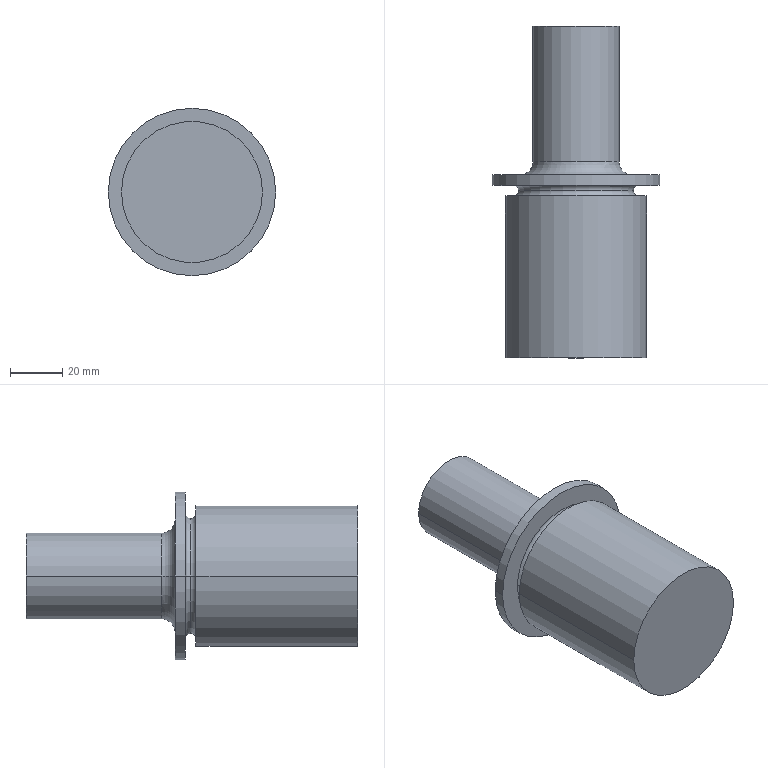Component | SolidWorks | Assembly4.1-1_114.1-1 | 1 solid | 17 faces | box 64 x 127 x 64 mm | volume 210532 mm3 | torus 6 | cylinder 6 | plane 5 | commonest cylinder face diameters 54 x2 64 x2 33 x2
STEP:
#1=CARTESIAN_POINT('',(-0.9449,-1.555,-0.01575));
#2=VERTEX_POINT('',#1);
#3=CARTESIAN_POINT('',(0.9449,-1.555,-0.01575));
#4=VERTEX_POINT('',#3);
#5=CARTESIAN_POINT('',(-0.,-1.555,-0.01575));
#6=DIRECTION('',(-0.,-1.,0.));
#7=DIRECTION('',(1.,0.,0.));
#8=AXIS2_PLACEMENT_3D('',#5,#6,#7);
#9=CIRCLE('',#8,0.9449);
#10=EDGE_CURVE('',#2,#4,#9,.T.);
#11=ORIENTED_EDGE('',*,*,#10,.F.);
#12=CARTESIAN_POINT('',(-0.8661,-1.476,-0.01575));
#13=VERTEX_POINT('',#12);
#14=CARTESIAN_POINT('',(-0.9449,-1.476,-0.01575));
#15=DIRECTION('',(-0.,0.,1.));
#16=DIRECTION('',(1.,0.,0.));
#17=AXIS2_PLACEMENT_3D('',#14,#15,#16);
#18=CIRCLE('',#17,0.07874);
#19=EDGE_CURVE('',#2,#13,#18,.T.);
#20=ORIENTED_EDGE('',*,*,#19,.T.);
#21=CARTESIAN_POINT('',(0.8661,-1.476,-0.01575));
#22=VERTEX_POINT('',#21);
#23=CARTESIAN_POINT('',(-0.,-1.476,-0.01575));
#24=DIRECTION('',(-0.,-1.,0.));
#25=DIRECTION('',(1.,0.,0.));
#26=AXIS2_PLACEMENT_3D('',#23,#24,#25);
#27=CIRCLE('',#26,0.8661);
#28=EDGE_CURVE('',#13,#22,#27,.T.);
#29=ORIENTED_EDGE('',*,*,#28,.T.);
#30=CARTESIAN_POINT('',(0.9449,-1.476,-0.01575));
#31=DIRECTION('',(0.,-0.,-1.));
#32=DIRECTION('',(-1.,0.,-0.));
#33=AXIS2_PLACEMENT_3D('',#30,#31,#32);
#34=CIRCLE('',#33,0.07874);
#35=EDGE_CURVE('',#4,#22,#34,.T.);
#36=ORIENTED_EDGE('',*,*,#35,.F.);
#37=EDGE_LOOP('',(#11,#20,#29,#36));
#38=FACE_OUTER_BOUND('',#37,.T.);
#39=CARTESIAN_POINT('',(-0.,-1.476,-0.01575));
#40=DIRECTION('',(-0.,-1.,0.));
#41=DIRECTION('',(1.,-0.,0.));
#42=AXIS2_PLACEMENT_3D('',#39,#40,#41);
#43=TOROIDAL_SURFACE('',#42,0.9449,0.07874);
#44=ADVANCED_FACE('',(#38),#43,.F.);
#45=ORIENTED_EDGE('',*,*,#28,.F.);
#46=CARTESIAN_POINT('',(-0.9449,-1.398,-0.01575));
#47=VERTEX_POINT('',#46);
#48=CARTESIAN_POINT('',(-0.9449,-1.476,-0.01575));
#49=DIRECTION('',(-0.,0.,1.));
#50=DIRECTION('',(1.,0.,0.));
#51=AXIS2_PLACEMENT_3D('',#48,#49,#50);
#52=CIRCLE('',#51,0.07874);
#53=EDGE_CURVE('',#13,#47,#52,.T.);
#54=ORIENTED_EDGE('',*,*,#53,.T.);
#55=CARTESIAN_POINT('',(0.9449,-1.398,-0.01575));
#56=VERTEX_POINT('',#55);
#57=CARTESIAN_POINT('',(-0.,-1.398,-0.01575));
#58=DIRECTION('',(0.,1.,-0.));
#59=DIRECTION('',(1.,0.,0.));
#60=AXIS2_PLACEMENT_3D('',#57,#58,#59);
#61=CIRCLE('',#60,0.9449);
#62=EDGE_CURVE('',#56,#47,#61,.T.);
#63=ORIENTED_EDGE('',*,*,#62,.F.);
#64=CARTESIAN_POINT('',(0.9449,-1.476,-0.01575));
#65=DIRECTION('',(0.,-0.,-1.));
#66=DIRECTION('',(-1.,0.,-0.));
#67=AXIS2_PLACEMENT_3D('',#64,#65,#66);
#68=CIRCLE('',#67,0.07874);
#69=EDGE_CURVE('',#22,#56,#68,.T.);
#70=ORIENTED_EDGE('',*,*,#69,.F.);
#71=EDGE_LOOP('',(#45,#54,#63,#70));
#72=FACE_OUTER_BOUND('',#71,.T.);
#73=CARTESIAN_POINT('',(-0.,-1.476,-0.01575));
#74=DIRECTION('',(-0.,-1.,0.));
#75=DIRECTION('',(1.,-0.,0.));
#76=AXIS2_PLACEMENT_3D('',#73,#74,#75);
#77=TOROIDAL_SURFACE('',#76,0.9449,0.07874);
#78=ADVANCED_FACE('',(#72),#77,.F.);
#79=CARTESIAN_POINT('',(1.063,-3.996,-0.01575));
#80=VERTEX_POINT('',#79);
#81=CARTESIAN_POINT('',(-1.063,-3.996,-0.01575));
#82=VERTEX_POINT('',#81);
#83=CARTESIAN_POINT('',(-0.,-3.996,-0.01575));
#84=DIRECTION('',(-0.,-1.,0.));
#85=DIRECTION('',(1.,0.,0.));
#86=AXIS2_PLACEMENT_3D('',#83,#84,#85);
#87=CIRCLE('',#86,1.063);
#88=EDGE_CURVE('',#80,#82,#87,.T.);
#89=ORIENTED_EDGE('',*,*,#88,.F.);
#90=CARTESIAN_POINT('',(1.063,-1.555,-0.01575));
#91=VERTEX_POINT('',#90);
#92=CARTESIAN_POINT('',(1.063,-3.996,-0.01575));
#93=DIRECTION('',(0.,1.,-0.));
#94=VECTOR('',#93,39.37);
#95=LINE('',#92,#94);
#96=EDGE_CURVE('',#80,#91,#95,.T.);
#97=ORIENTED_EDGE('',*,*,#96,.T.);
#98=CARTESIAN_POINT('',(-1.063,-1.555,-0.01575));
#99=VERTEX_POINT('',#98);
#100=CARTESIAN_POINT('',(-0.,-1.555,-0.01575));
#101=DIRECTION('',(-0.,-1.,0.));
#102=DIRECTION('',(1.,0.,0.));
#103=AXIS2_PLACEMENT_3D('',#100,#101,#102);
#104=CIRCLE('',#103,1.063);
#105=EDGE_CURVE('',#91,#99,#104,.T.);
#106=ORIENTED_EDGE('',*,*,#105,.T.);
#107=CARTESIAN_POINT('',(-1.063,-3.996,-0.01575));
#108=DIRECTION('',(0.,1.,-0.));
#109=VECTOR('',#108,39.37);
#110=LINE('',#107,#109);
#111=EDGE_CURVE('',#82,#99,#110,.T.);
#112=ORIENTED_EDGE('',*,*,#111,.F.);
#113=EDGE_LOOP('',(#89,#97,#106,#112));
#114=FACE_OUTER_BOUND('',#113,.T.);
#115=CARTESIAN_POINT('',(-0.,-3.996,-0.01575));
#116=DIRECTION('',(0.,1.,-0.));
#117=DIRECTION('',(-1.,0.,-0.));
#118=AXIS2_PLACEMENT_3D('',#115,#116,#117);
#119=CYLINDRICAL_SURFACE('',#118,1.063);
#120=ADVANCED_FACE('',(#114),#119,.T.);
#121=CARTESIAN_POINT('',(-0.8465,-1.24,-0.01575));
#122=VERTEX_POINT('',#121);
#123=CARTESIAN_POINT('',(0.8465,-1.24,-0.01575));
#124=VERTEX_POINT('',#123);
#125=CARTESIAN_POINT('',(-0.,-1.24,-0.01575));
#126=DIRECTION('',(-0.,-1.,0.));
#127=DIRECTION('',(1.,0.,0.));
#128=AXIS2_PLACEMENT_3D('',#125,#126,#127);
#129=CIRCLE('',#128,0.8465);
#130=EDGE_CURVE('',#122,#124,#129,.T.);
#131=ORIENTED_EDGE('',*,*,#130,.F.);
#132=CARTESIAN_POINT('',(-0.6496,-1.043,-0.01575));
#133=VERTEX_POINT('',#132);
#134=CARTESIAN_POINT('',(-0.8465,-1.043,-0.01575));
#135=DIRECTION('',(-0.,0.,1.));
#136=DIRECTION('',(1.,0.,0.));
#137=AXIS2_PLACEMENT_3D('',#134,#135,#136);
#138=CIRCLE('',#137,0.1969);
#139=EDGE_CURVE('',#122,#133,#138,.T.);
#140=ORIENTED_EDGE('',*,*,#139,.T.);
#141=CARTESIAN_POINT('',(0.6496,-1.043,-0.01575));
#142=VERTEX_POINT('',#141);
#143=CARTESIAN_POINT('',(-0.,-1.043,-0.01575));
#144=DIRECTION('',(0.,1.,-0.));
#145=DIRECTION('',(1.,0.,0.));
#146=AXIS2_PLACEMENT_3D('',#143,#144,#145);
#147=CIRCLE('',#146,0.6496);
#148=EDGE_CURVE('',#142,#133,#147,.T.);
#149=ORIENTED_EDGE('',*,*,#148,.F.);
#150=CARTESIAN_POINT('',(0.8465,-1.043,-0.01575));
#151=DIRECTION('',(0.,-0.,-1.));
#152=DIRECTION('',(-1.,0.,-0.));
#153=AXIS2_PLACEMENT_3D('',#150,#151,#152);
#154=CIRCLE('',#153,0.1969);
#155=EDGE_CURVE('',#124,#142,#154,.T.);
#156=ORIENTED_EDGE('',*,*,#155,.F.);
#157=EDGE_LOOP('',(#131,#140,#149,#156));
#158=FACE_OUTER_BOUND('',#157,.T.);
#159=CARTESIAN_POINT('',(-0.,-1.043,-0.01575));
#160=DIRECTION('',(-0.,-1.,0.));
#161=DIRECTION('',(1.,-0.,0.));
#162=AXIS2_PLACEMENT_3D('',#159,#160,#161);
#163=TOROIDAL_SURFACE('',#162,0.8465,0.1969);
#164=ADVANCED_FACE('',(#158),#163,.F.);
#165=CARTESIAN_POINT('',(1.26,-1.398,-0.01575));
#166=VERTEX_POINT('',#165);
#167=CARTESIAN_POINT('',(-1.26,-1.398,-0.01575));
#168=VERTEX_POINT('',#167);
#169=CARTESIAN_POINT('',(-0.,-1.398,-0.01575));
#170=DIRECTION('',(-0.,-1.,0.));
#171=DIRECTION('',(1.,0.,0.));
#172=AXIS2_PLACEMENT_3D('',#169,#170,#171);
#173=CIRCLE('',#172,1.26);
#174=EDGE_CURVE('',#166,#168,#173,.T.);
#175=ORIENTED_EDGE('',*,*,#174,.F.);
#176=CARTESIAN_POINT('',(1.26,-1.24,-0.01575));
#177=VERTEX_POINT('',#176);
#178=CARTESIAN_POINT('',(1.26,-1.398,-0.01575));
#179=DIRECTION('',(0.,1.,-0.));
#180=VECTOR('',#179,39.37);
#181=LINE('',#178,#180);
#182=EDGE_CURVE('',#166,#177,#181,.T.);
#183=ORIENTED_EDGE('',*,*,#182,.T.);
#184=CARTESIAN_POINT('',(-1.26,-1.24,-0.01575));
#185=VERTEX_POINT('',#184);
#186=CARTESIAN_POINT('',(-0.,-1.24,-0.01575));
#187=DIRECTION('',(-0.,-1.,0.));
#188=DIRECTION('',(1.,0.,0.));
#189=AXIS2_PLACEMENT_3D('',#186,#187,#188);
#190=CIRCLE('',#189,1.26);
#191=EDGE_CURVE('',#177,#185,#190,.T.);
#192=ORIENTED_EDGE('',*,*,#191,.T.);
#193=CARTESIAN_POINT('',(-1.26,-1.398,-0.01575));
#194=DIRECTION('',(0.,1.,-0.));
#195=VECTOR('',#194,39.37);
#196=LINE('',#193,#195);
#197=EDGE_CURVE('',#168,#185,#196,.T.);
#198=ORIENTED_EDGE('',*,*,#197,.F.);
#199=EDGE_LOOP('',(#175,#183,#192,#198));
#200=FACE_OUTER_BOUND('',#199,.T.);
#201=CARTESIAN_POINT('',(-0.,-1.398,-0.01575));
#202=DIRECTION('',(0.,1.,-0.));
#203=DIRECTION('',(-1.,0.,-0.));
#204=AXIS2_PLACEMENT_3D('',#201,#202,#203);
#205=CYLINDRICAL_SURFACE('',#204,1.26);
#206=ADVANCED_FACE('',(#200),#205,.T.);
#207=CARTESIAN_POINT('',(-0.6496,1.004,-0.01575));
#208=VERTEX_POINT('',#207);
#209=CARTESIAN_POINT('',(0.6496,1.004,-0.01575));
#210=VERTEX_POINT('',#209);
#211=CARTESIAN_POINT('',(0.,1.004,-0.01575));
#212=DIRECTION('',(0.,1.,-0.));
#213=DIRECTION('',(-1.,0.,-0.));
#214=AXIS2_PLACEMENT_3D('',#211,#212,#213);
#215=CIRCLE('',#214,0.6496);
#216=EDGE_CURVE('',#208,#210,#215,.T.);
#217=ORIENTED_EDGE('',*,*,#216,.F.);
#218=CARTESIAN_POINT('',(-0.6496,1.004,-0.01575));
#219=DIRECTION('',(-0.,-1.,0.));
#220=VECTOR('',#219,39.37);
#221=LINE('',#218,#220);
#222=EDGE_CURVE('',#208,#133,#221,.T.);
#223=ORIENTED_EDGE('',*,*,#222,.T.);
#224=CARTESIAN_POINT('',(-0.,-1.043,-0.01575));
#225=DIRECTION('',(0.,1.,-0.));
#226=DIRECTION('',(1.,0.,0.));
#227=AXIS2_PLACEMENT_3D('',#224,#225,#226);
#228=CIRCLE('',#227,0.6496);
#229=EDGE_CURVE('',#133,#142,#228,.T.);
#230=ORIENTED_EDGE('',*,*,#229,.T.);
#231=CARTESIAN_POINT('',(0.6496,1.004,-0.01575));
#232=DIRECTION('',(-0.,-1.,0.));
#233=VECTOR('',#232,39.37);
#234=LINE('',#231,#233);
#235=EDGE_CURVE('',#210,#142,#234,.T.);
#236=ORIENTED_EDGE('',*,*,#235,.F.);
#237=EDGE_LOOP('',(#217,#223,#230,#236));
#238=FACE_OUTER_BOUND('',#237,.T.);
#239=CARTESIAN_POINT('',(0.,1.004,-0.01575));
#240=DIRECTION('',(-0.,-1.,0.));
#241=DIRECTION('',(1.,0.,0.));
#242=AXIS2_PLACEMENT_3D('',#239,#240,#241);
#243=CYLINDRICAL_SURFACE('',#242,0.6496);
#244=ADVANCED_FACE('',(#238),#243,.T.);
#245=ORIENTED_EDGE('',*,*,#62,.T.);
#246=CARTESIAN_POINT('',(-0.,-1.398,-0.01575));
#247=DIRECTION('',(0.,1.,-0.));
#248=DIRECTION('',(1.,0.,0.));
#249=AXIS2_PLACEMENT_3D('',#246,#247,#248);
#250=CIRCLE('',#249,0.9449);
#251=EDGE_CURVE('',#47,#56,#250,.T.);
#252=ORIENTED_EDGE('',*,*,#251,.T.);
#253=EDGE_LOOP('',(#245,#252));
#254=FACE_BOUND('',#253,.T.);
#255=CARTESIAN_POINT('',(-0.,-1.398,-0.01575));
#256=DIRECTION('',(-0.,-1.,0.));
#257=DIRECTION('',(1.,0.,0.));
#258=AXIS2_PLACEMENT_3D('',#255,#256,#257);
#259=CIRCLE('',#258,1.26);
#260=EDGE_CURVE('',#168,#166,#259,.T.);
#261=ORIENTED_EDGE('',*,*,#260,.T.);
#262=ORIENTED_EDGE('',*,*,#174,.T.);
#263=EDGE_LOOP('',(#261,#262));
#264=FACE_OUTER_BOUND('',#263,.T.);
#265=CARTESIAN_POINT('',(-0.,-1.398,-0.01575));
#266=DIRECTION('',(-0.,-1.,0.));
#267=DIRECTION('',(1.,-0.,0.));
#268=AXIS2_PLACEMENT_3D('',#265,#266,#267);
#269=PLANE('',#268);
#270=ADVANCED_FACE('',(#254,#264),#269,.T.);
#271=ORIENTED_EDGE('',*,*,#222,.F.);
#272=CARTESIAN_POINT('',(0.,1.004,-0.01575));
#273=DIRECTION('',(0.,1.,-0.));
#274=DIRECTION('',(-1.,0.,-0.));
#275=AXIS2_PLACEMENT_3D('',#272,#273,#274);
#276=CIRCLE('',#275,0.6496);
#277=EDGE_CURVE('',#210,#208,#276,.T.);
#278=ORIENTED_EDGE('',*,*,#277,.F.);
#279=ORIENTED_EDGE('',*,*,#235,.T.);
#280=ORIENTED_EDGE('',*,*,#148,.T.);
#281=EDGE_LOOP('',(#271,#278,#279,#280));
#282=FACE_OUTER_BOUND('',#281,.T.);
#283=CARTESIAN_POINT('',(0.,1.004,-0.01575));
#284=DIRECTION('',(-0.,-1.,0.));
#285=DIRECTION('',(1.,0.,0.));
#286=AXIS2_PLACEMENT_3D('',#283,#284,#285);
#287=CYLINDRICAL_SURFACE('',#286,0.6496);
#288=ADVANCED_FACE('',(#282),#287,.T.);
#289=ORIENTED_EDGE('',*,*,#277,.T.);
#290=ORIENTED_EDGE('',*,*,#216,.T.);
#291=EDGE_LOOP('',(#289,#290));
#292=FACE_OUTER_BOUND('',#291,.T.);
#293=CARTESIAN_POINT('',(0.,1.004,-0.01575));
#294=DIRECTION('',(0.,1.,-0.));
#295=DIRECTION('',(-1.,0.,-0.));
#296=AXIS2_PLACEMENT_3D('',#293,#294,#295);
#297=PLANE('',#296);
#298=ADVANCED_FACE('',(#292),#297,.T.);
#299=CARTESIAN_POINT('',(-0.,-1.24,-0.01575));
#300=DIRECTION('',(-0.,-1.,0.));
#301=DIRECTION('',(1.,0.,0.));
#302=AXIS2_PLACEMENT_3D('',#299,#300,#301);
#303=CIRCLE('',#302,0.8465);
#304=EDGE_CURVE('',#124,#122,#303,.T.);
#305=ORIENTED_EDGE('',*,*,#304,.T.);
#306=ORIENTED_EDGE('',*,*,#130,.T.);
#307=EDGE_LOOP('',(#305,#306));
#308=FACE_BOUND('',#307,.T.);
#309=CARTESIAN_POINT('',(-0.,-1.24,-0.01575));
#310=DIRECTION('',(-0.,-1.,0.));
#311=DIRECTION('',(1.,0.,0.));
#312=AXIS2_PLACEMENT_3D('',#309,#310,#311);
#313=CIRCLE('',#312,1.26);
#314=EDGE_CURVE('',#185,#177,#313,.T.);
#315=ORIENTED_EDGE('',*,*,#314,.F.);
#316=ORIENTED_EDGE('',*,*,#191,.F.);
#317=EDGE_LOOP('',(#315,#316));
#318=FACE_OUTER_BOUND('',#317,.T.);
#319=CARTESIAN_POINT('',(-0.,-1.24,-0.01575));
#320=DIRECTION('',(-0.,-1.,0.));
#321=DIRECTION('',(1.,-0.,0.));
#322=AXIS2_PLACEMENT_3D('',#319,#320,#321);
#323=PLANE('',#322);
#324=ADVANCED_FACE('',(#308,#318),#323,.F.);
#325=ORIENTED_EDGE('',*,*,#182,.F.);
#326=ORIENTED_EDGE('',*,*,#260,.F.);
#327=ORIENTED_EDGE('',*,*,#197,.T.);
#328=ORIENTED_EDGE('',*,*,#314,.T.);
#329=EDGE_LOOP('',(#325,#326,#327,#328));
#330=FACE_OUTER_BOUND('',#329,.T.);
#331=CARTESIAN_POINT('',(-0.,-1.398,-0.01575));
#332=DIRECTION('',(0.,1.,-0.));
#333=DIRECTION('',(-1.,0.,-0.));
#334=AXIS2_PLACEMENT_3D('',#331,#332,#333);
#335=CYLINDRICAL_SURFACE('',#334,1.26);
#336=ADVANCED_FACE('',(#330),#335,.T.);
#337=ORIENTED_EDGE('',*,*,#139,.F.);
#338=ORIENTED_EDGE('',*,*,#304,.F.);
#339=ORIENTED_EDGE('',*,*,#155,.T.);
#340=ORIENTED_EDGE('',*,*,#229,.F.);
#341=EDGE_LOOP('',(#337,#338,#339,#340));
#342=FACE_OUTER_BOUND('',#341,.T.);
#343=CARTESIAN_POINT('',(-0.,-1.043,-0.01575));
#344=DIRECTION('',(-0.,-1.,0.));
#345=DIRECTION('',(1.,-0.,0.));
#346=AXIS2_PLACEMENT_3D('',#343,#344,#345);
#347=TOROIDAL_SURFACE('',#346,0.8465,0.1969);
#348=ADVANCED_FACE('',(#342),#347,.F.);
#349=CARTESIAN_POINT('',(-0.,-1.555,-0.01575));
#350=DIRECTION('',(-0.,-1.,0.));
#351=DIRECTION('',(1.,0.,0.));
#352=AXIS2_PLACEMENT_3D('',#349,#350,#351);
#353=CIRCLE('',#352,0.9449);
#354=EDGE_CURVE('',#4,#2,#353,.T.);
#355=ORIENTED_EDGE('',*,*,#354,.T.);
#356=ORIENTED_EDGE('',*,*,#10,.T.);
#357=EDGE_LOOP('',(#355,#356));
#358=FACE_BOUND('',#357,.T.);
#359=CARTESIAN_POINT('',(-0.,-1.555,-0.01575));
#360=DIRECTION('',(-0.,-1.,0.));
#361=DIRECTION('',(1.,0.,0.));
#362=AXIS2_PLACEMENT_3D('',#359,#360,#361);
#363=CIRCLE('',#362,1.063);
#364=EDGE_CURVE('',#99,#91,#363,.T.);
#365=ORIENTED_EDGE('',*,*,#364,.F.);
#366=ORIENTED_EDGE('',*,*,#105,.F.);
#367=EDGE_LOOP('',(#365,#366));
#368=FACE_OUTER_BOUND('',#367,.T.);
#369=CARTESIAN_POINT('',(-0.,-1.555,-0.01575));
#370=DIRECTION('',(-0.,-1.,0.));
#371=DIRECTION('',(1.,-0.,0.));
#372=AXIS2_PLACEMENT_3D('',#369,#370,#371);
#373=PLANE('',#372);
#374=ADVANCED_FACE('',(#358,#368),#373,.F.);
#375=ORIENTED_EDGE('',*,*,#96,.F.);
#376=CARTESIAN_POINT('',(-0.,-3.996,-0.01575));
#377=DIRECTION('',(-0.,-1.,0.));
#378=DIRECTION('',(1.,0.,0.));
#379=AXIS2_PLACEMENT_3D('',#376,#377,#378);
#380=CIRCLE('',#379,1.063);
#381=EDGE_CURVE('',#82,#80,#380,.T.);
#382=ORIENTED_EDGE('',*,*,#381,.F.);
#383=ORIENTED_EDGE('',*,*,#111,.T.);
#384=ORIENTED_EDGE('',*,*,#364,.T.);
#385=EDGE_LOOP('',(#375,#382,#383,#384));
#386=FACE_OUTER_BOUND('',#385,.T.);
#387=CARTESIAN_POINT('',(-0.,-3.996,-0.01575));
#388=DIRECTION('',(0.,1.,-0.));
#389=DIRECTION('',(-1.,0.,-0.));
#390=AXIS2_PLACEMENT_3D('',#387,#388,#389);
#391=CYLINDRICAL_SURFACE('',#390,1.063);
#392=ADVANCED_FACE('',(#386),#391,.T.);
#393=ORIENTED_EDGE('',*,*,#381,.T.);
#394=ORIENTED_EDGE('',*,*,#88,.T.);
#395=EDGE_LOOP('',(#393,#394));
#396=FACE_OUTER_BOUND('',#395,.T.);
#397=CARTESIAN_POINT('',(-0.,-3.996,-0.01575));
#398=DIRECTION('',(-0.,-1.,0.));
#399=DIRECTION('',(1.,-0.,0.));
#400=AXIS2_PLACEMENT_3D('',#397,#398,#399);
#401=PLANE('',#400);
#402=ADVANCED_FACE('',(#396),#401,.T.);
#403=ORIENTED_EDGE('',*,*,#53,.F.);
#404=CARTESIAN_POINT('',(-0.,-1.476,-0.01575));
#405=DIRECTION('',(-0.,-1.,0.));
#406=DIRECTION('',(1.,0.,0.));
#407=AXIS2_PLACEMENT_3D('',#404,#405,#406);
#408=CIRCLE('',#407,0.8661);
#409=EDGE_CURVE('',#22,#13,#408,.T.);
#410=ORIENTED_EDGE('',*,*,#409,.F.);
#411=ORIENTED_EDGE('',*,*,#69,.T.);
#412=ORIENTED_EDGE('',*,*,#251,.F.);
#413=EDGE_LOOP('',(#403,#410,#411,#412));
#414=FACE_OUTER_BOUND('',#413,.T.);
#415=CARTESIAN_POINT('',(-0.,-1.476,-0.01575));
#416=DIRECTION('',(-0.,-1.,0.));
#417=DIRECTION('',(1.,-0.,0.));
#418=AXIS2_PLACEMENT_3D('',#415,#416,#417);
#419=TOROIDAL_SURFACE('',#418,0.9449,0.07874);
#420=ADVANCED_FACE('',(#414),#419,.F.);
#421=ORIENTED_EDGE('',*,*,#19,.F.);
#422=ORIENTED_EDGE('',*,*,#354,.F.);
#423=ORIENTED_EDGE('',*,*,#35,.T.);
#424=ORIENTED_EDGE('',*,*,#409,.T.);
#425=EDGE_LOOP('',(#421,#422,#423,#424));
#426=FACE_OUTER_BOUND('',#425,.T.);
#427=CARTESIAN_POINT('',(-0.,-1.476,-0.01575));
#428=DIRECTION('',(-0.,-1.,0.));
#429=DIRECTION('',(1.,-0.,0.));
#430=AXIS2_PLACEMENT_3D('',#427,#428,#429);
#431=TOROIDAL_SURFACE('',#430,0.9449,0.07874);
#432=ADVANCED_FACE('',(#426),#431,.F.);
#433=CLOSED_SHELL('',(#44,#78,#120,#164,#206,#244,#270,#288,#298,#324,#336,#348,#374,#392,#402,#420,#432));
#434=MANIFOLD_SOLID_BREP('',#433);
#435=CARTESIAN_POINT('',(0.,0.,0.));
#436=DIRECTION('',(0.,0.,1.));
#437=DIRECTION('',(1.,0.,0.));
#438=AXIS2_PLACEMENT_3D('',#435,#436,#437);
#439=(LENGTH_UNIT()NAMED_UNIT(*)SI_UNIT($,.METRE.));
#440=LENGTH_MEASURE_WITH_UNIT(LENGTH_MEASURE(0.0254),#439);
#441=DIMENSIONAL_EXPONENTS(1.,0.,0.,0.,0.,0.,0.);
#442=(CONVERSION_BASED_UNIT('',#440)LENGTH_UNIT()NAMED_UNIT(#441));
#443=UNCERTAINTY_MEASURE_WITH_UNIT(LENGTH_MEASURE(0.00001),#442,'','');
#444=(NAMED_UNIT(*)PLANE_ANGLE_UNIT()SI_UNIT($,.RADIAN.));
#445=(NAMED_UNIT(*)SI_UNIT($,.STERADIAN.)SOLID_ANGLE_UNIT());
#446=(GEOMETRIC_REPRESENTATION_CONTEXT(3)GLOBAL_UNCERTAINTY_ASSIGNED_CONTEXT((#443))GLOBAL_UNIT_ASSIGNED_CONTEXT((#442,#444,#445))REPRESENTATION_CONTEXT('',''));
#447=ADVANCED_BREP_SHAPE_REPRESENTATION('',(#434,#438),#446);
#448=COLOUR_RGB('',0.7922,0.8196,0.9333);
#449=FILL_AREA_STYLE_COLOUR('',#448);
#450=FILL_AREA_STYLE('',(#449));
#451=SURFACE_STYLE_FILL_AREA(#450);
#452=SURFACE_SIDE_STYLE('',(#451));
#453=SURFACE_STYLE_USAGE(.BOTH.,#452);
#454=PRESENTATION_STYLE_ASSIGNMENT((#453));
#455=STYLED_ITEM('',(#454),#434);
#456=(LENGTH_UNIT()NAMED_UNIT(*)SI_UNIT($,.METRE.));
#457=LENGTH_MEASURE_WITH_UNIT(LENGTH_MEASURE(0.0254),#456);
#458=DIMENSIONAL_EXPONENTS(1.,0.,0.,0.,0.,0.,0.);
#459=(CONVERSION_BASED_UNIT('',#457)LENGTH_UNIT()NAMED_UNIT(#458));
#460=UNCERTAINTY_MEASURE_WITH_UNIT(LENGTH_MEASURE(0.00001),#459,'','');
#461=(NAMED_UNIT(*)PLANE_ANGLE_UNIT()SI_UNIT($,.RADIAN.));
#462=(NAMED_UNIT(*)SI_UNIT($,.STERADIAN.)SOLID_ANGLE_UNIT());
#463=(GEOMETRIC_REPRESENTATION_CONTEXT(3)GLOBAL_UNCERTAINTY_ASSIGNED_CONTEXT((#460))GLOBAL_UNIT_ASSIGNED_CONTEXT((#459,#461,#462))REPRESENTATION_CONTEXT('',''));
#464=MECHANICAL_DESIGN_GEOMETRIC_PRESENTATION_REPRESENTATION('',(#455),#463);
#465=PRESENTATION_LAYER_ASSIGNMENT('','',(#455));